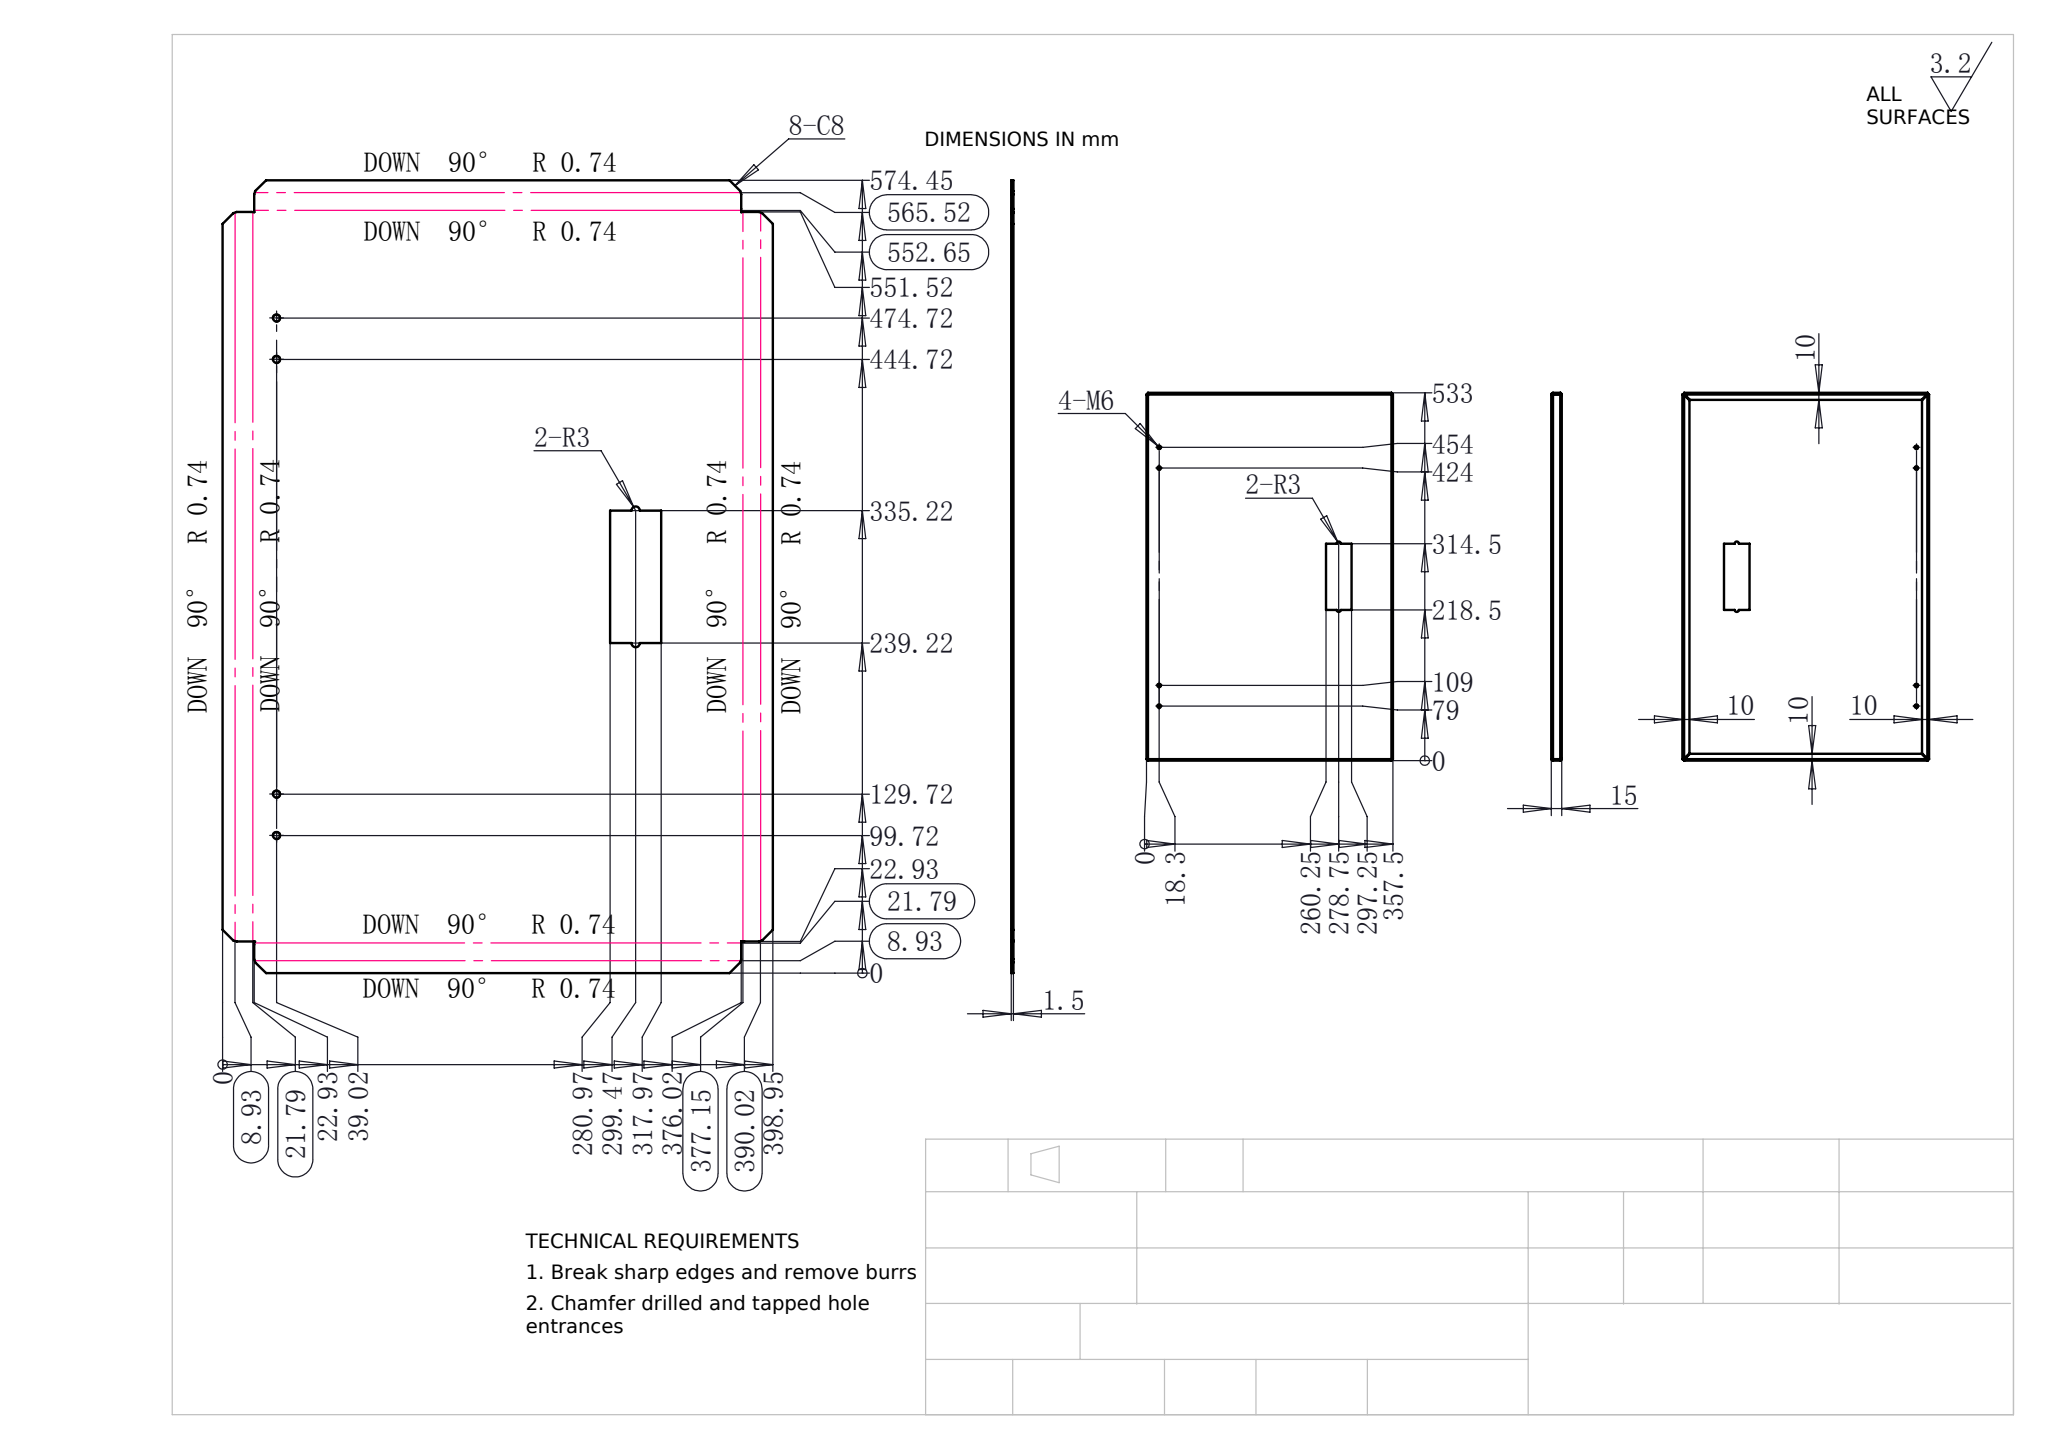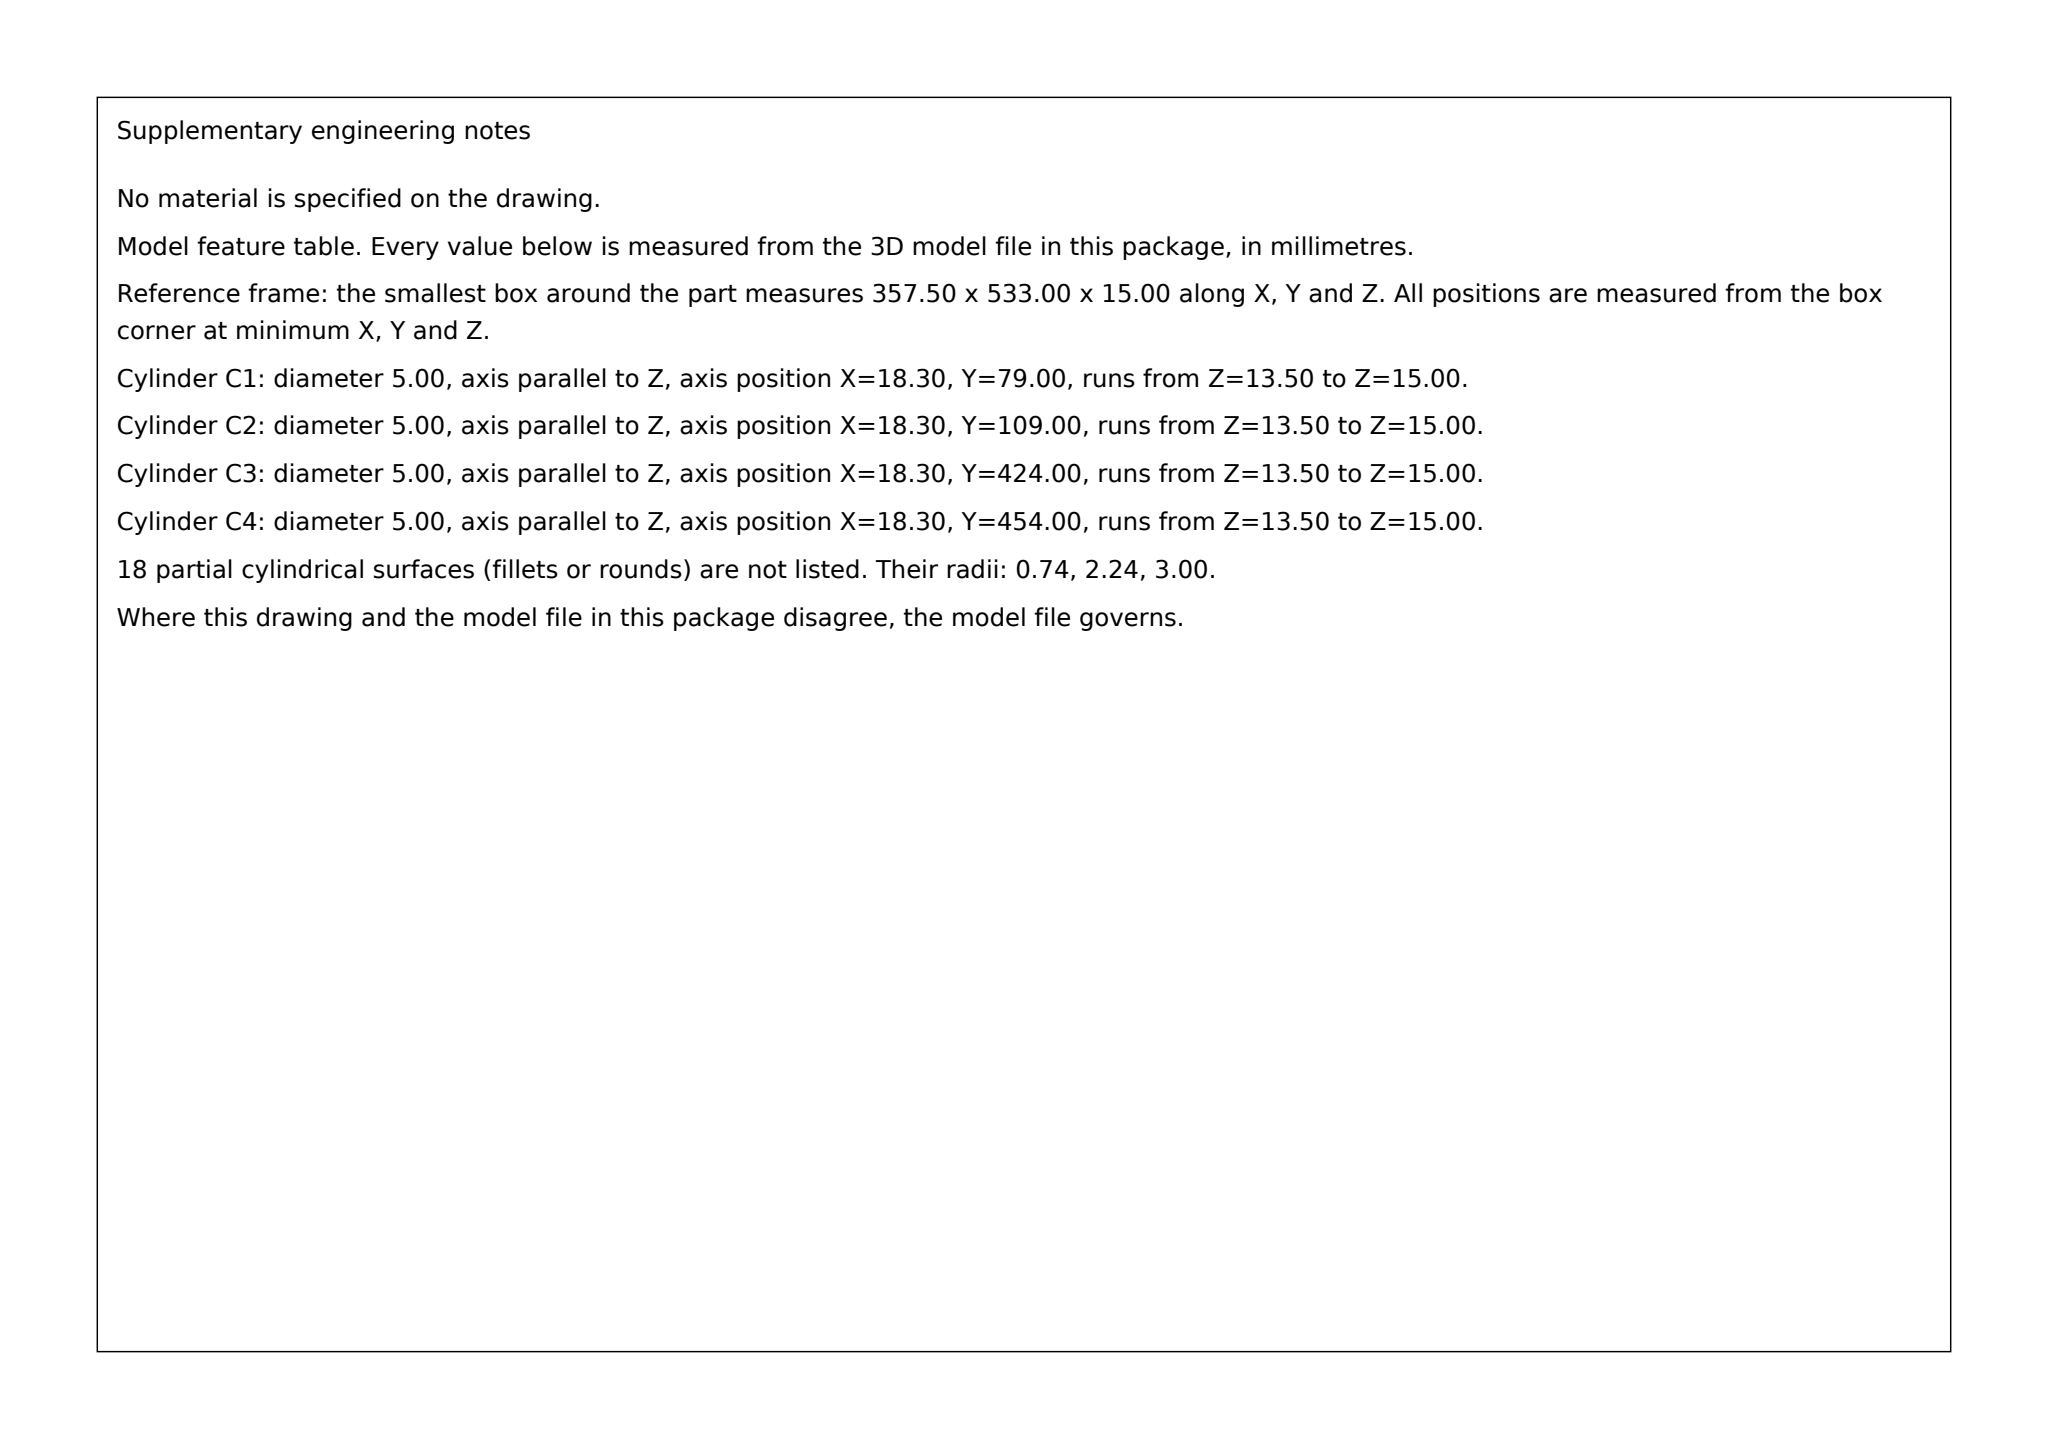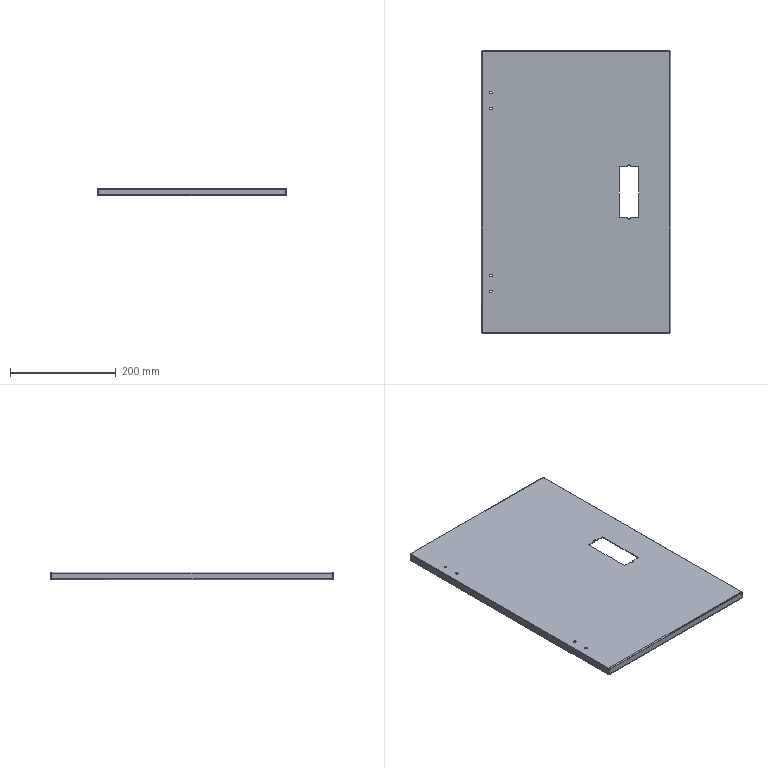Part | SolidWorks | mm | 1 solid | 86 faces | box 357.5 x 533 x 15 mm | volume 334678 mm3 | plane 44 | cylinder 26 | spline 16 | commonest cylinder face diameters 5 x8 4.473 x8 1.473 x8 6 x2